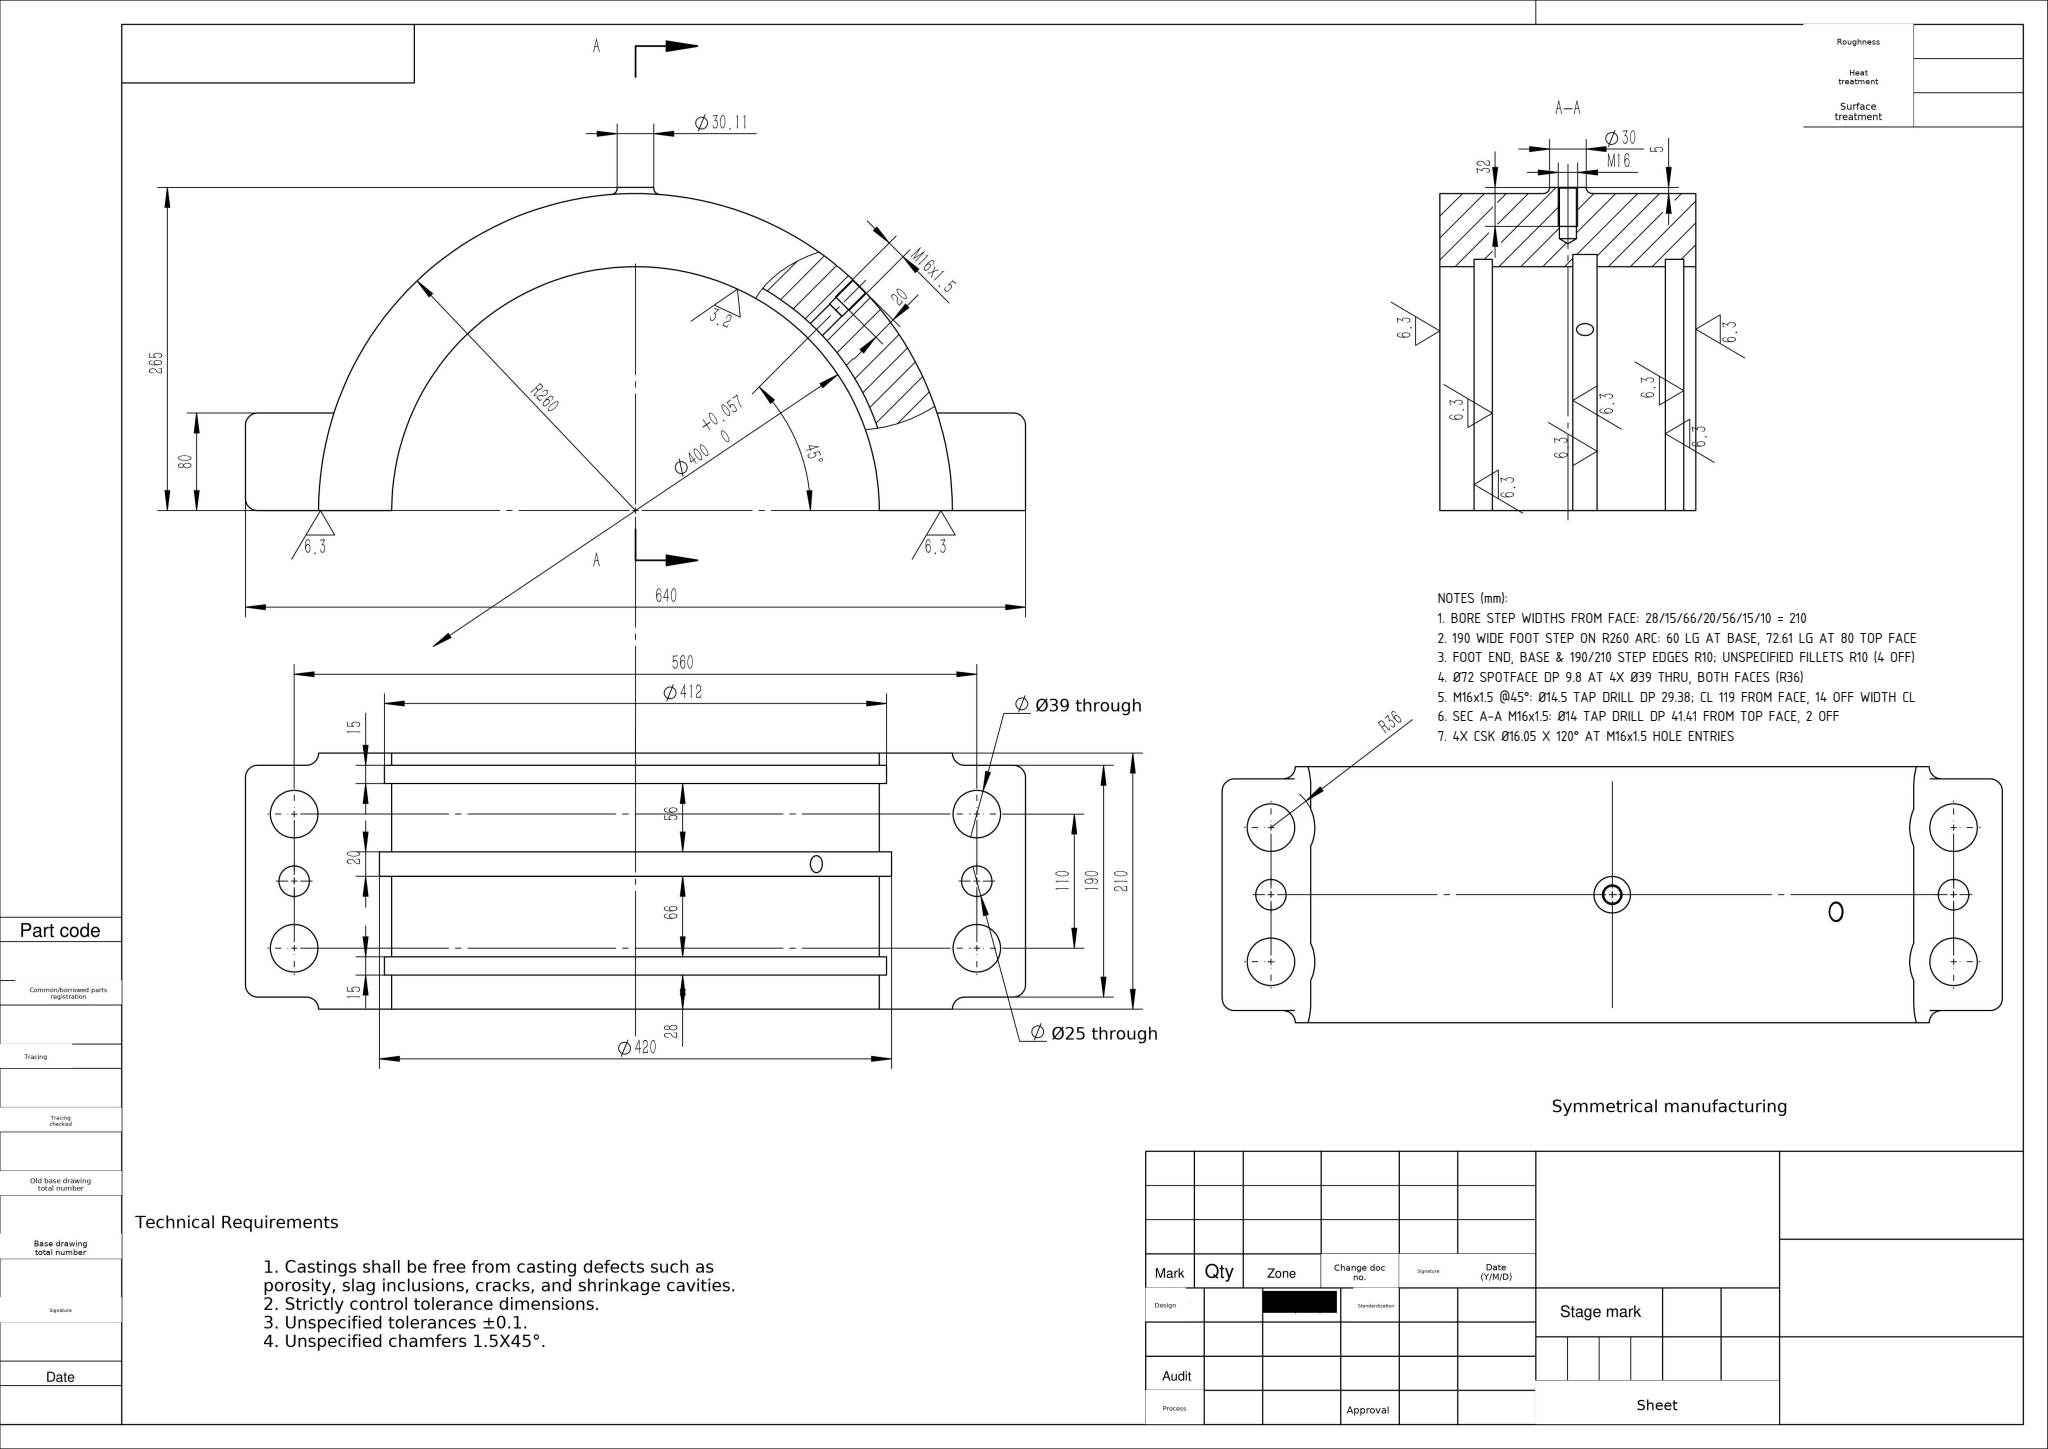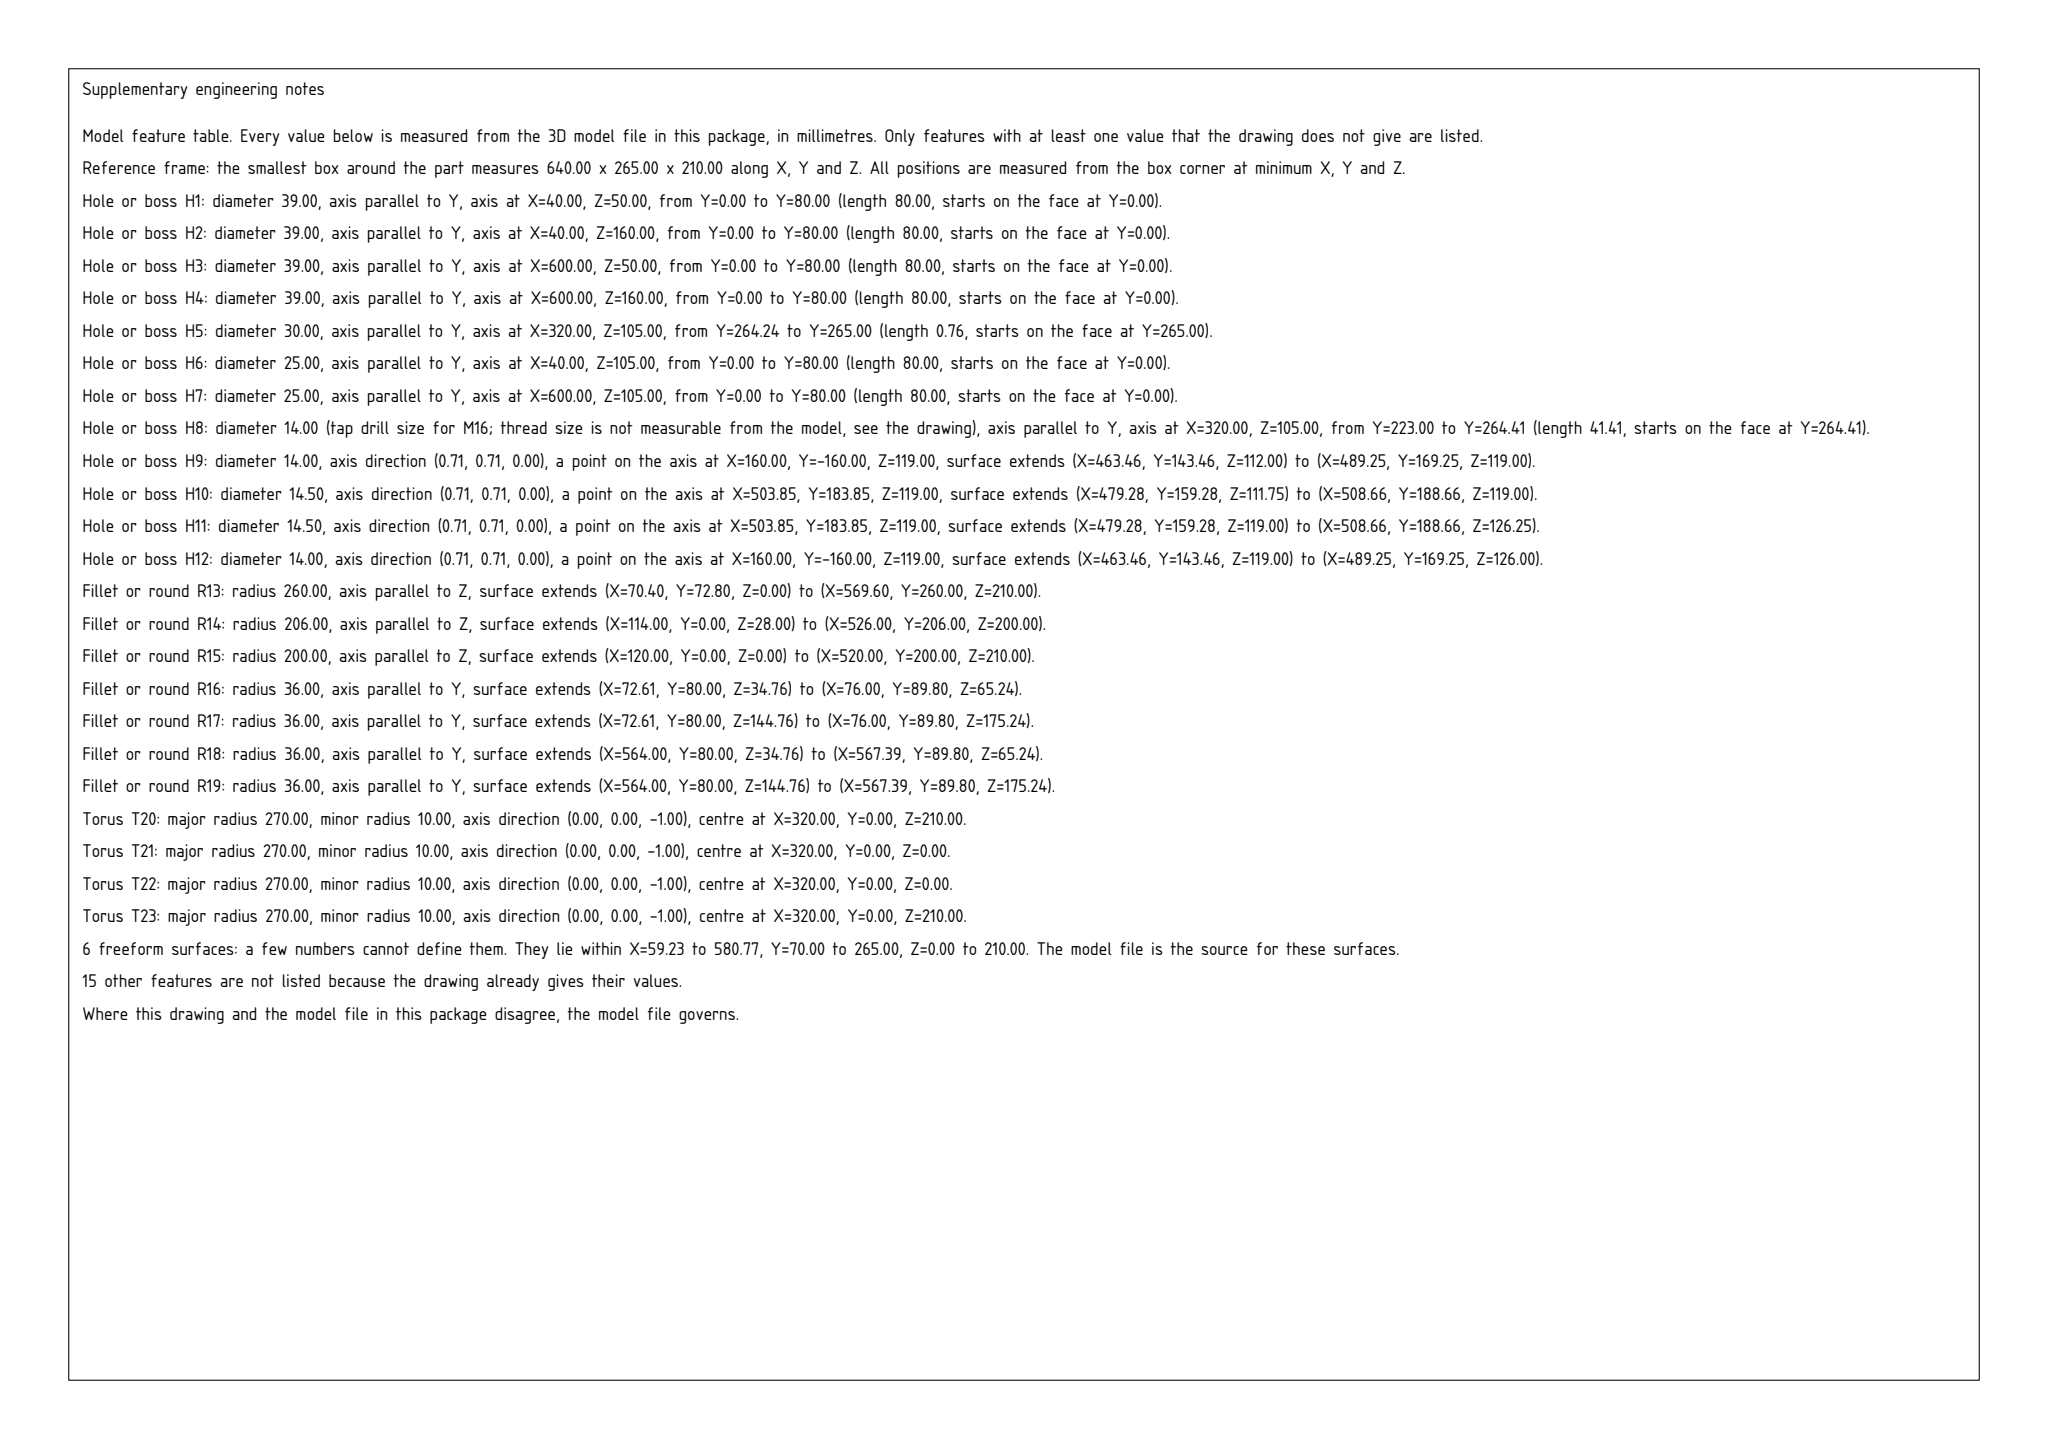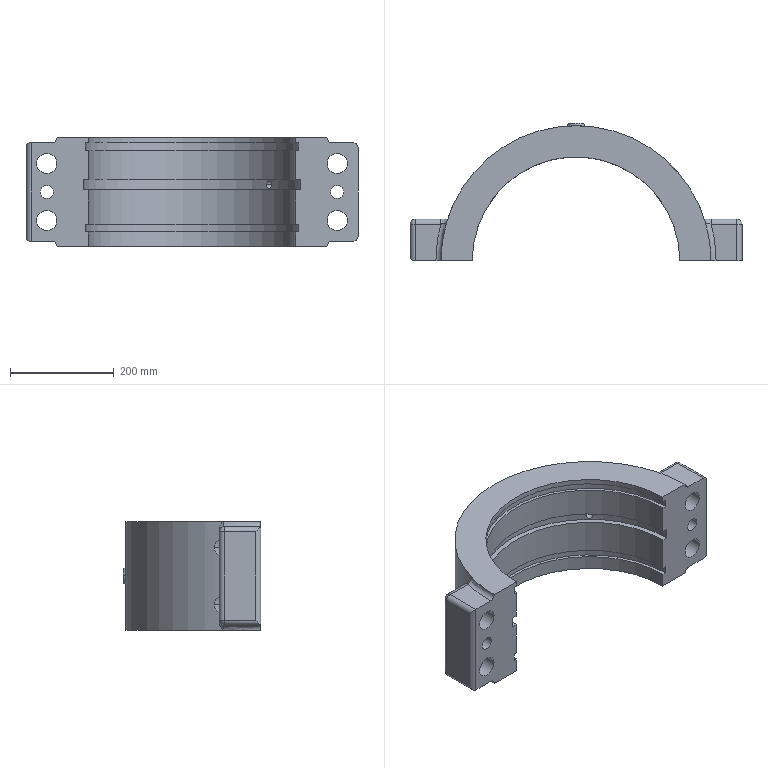Part | SolidWorks | mm | 1 solid | 87 faces | box 640 x 265 x 210 mm | volume 10321361 mm3 | cylinder 46 | plane 19 | cone 8 | spline 6 | torus 4 | sphere 4 | commonest cylinder face diameters 20 x11 39 x8 72 x6 14 x4 25 x4 400 x4 30 x3 14.5 x2
Drawing notes:
BORE STEP WIDTHS FROM FACE: 28/15/66/20/56/15/10 = 210 | from the solid: z-planes 0.19/28.19/43.19/109.19/129.19/185.19/200.19/210.19; Ø400 L28,66,56,10; Ø412 L15 x2; Ø420 L20
190 WIDE FOOT STEP ON R260 ARC: 60 LG AT BASE, 72.61 LG AT 80 TOP FACE | from the solid: Ø520 body axis z ctr x=320,y=0; foot top plane y=80; 320-260=60, 320-sqrt(260²-80²)=72.61; faces z=10.19/200.19 (190) vs 0.19/210.19 (210)
FOOT END, BASE & 190/210 STEP EDGES R10; UNSPECIFIED FILLETS R10 (4 OFF) | from the solid: fillet_radii [10.0,4]; Ø20 edge-round cyls: z-axis at (10,10),(10,70),(630,70); x-axis y=70 z=20.19/190.19 L49.23; y-axis x=10/630 z=20.19/190.19 L70
Ø72 SPOTFACE DP 9.8 AT 4X Ø39 THRU, BOTH FACES (R36) | from the solid: cyls dia 72 axis y at x=40/600, z=50.19/160.19, L9.8, coaxial with Ø39 thru holes
M16x1.5 @45°: Ø14.5 TAP DRILL DP 29.38; CL 119 FROM FACE, 14 OFF WIDTH CL | from the solid: cyl [14.5,'x',[null,183.85,119.19],29.38] with 118° point; 183.85=260/√2 (R260 at 45°); part z 0.19-210.19, CL 105.19
SEC A-A M16x1.5: Ø14 TAP DRILL DP 41.41 FROM TOP FACE, 2 OFF | from the solid: cyl dia 14.0 axis y at x=320, z=105.19, L41.41, 2 off; 118° drill point cone ref dia 14.0
4X CSK Ø16.05 X 120° AT M16x1.5 HOLE ENTRIES | from the solid: cones [120.0, 16.05, 4] at the four M16x1.5 holes (2X Ø14 axis x, 2X Ø14 axis y)